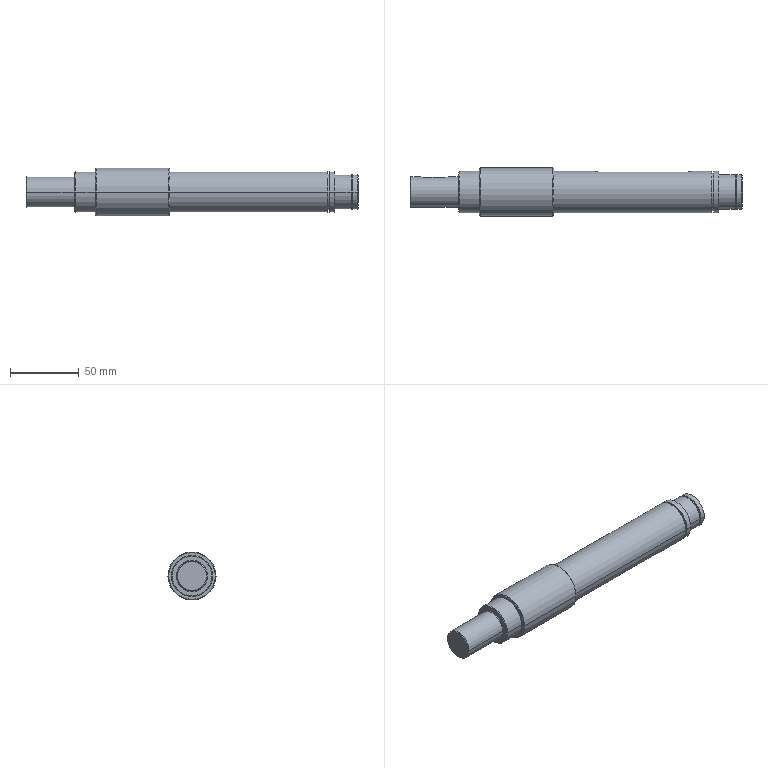Component | SolidWorks | LowerSideBeltXG-XG1-1_DrivePulleyDriveShaftXG-XG1-1 | 1 solid | 56 faces | box 241.5 x 35 x 35 mm | volume 165623 mm3 | cylinder 26 | plane 16 | cone 12 | torus 2 | commonest cylinder face diameters 30 x6 6 x5 25 x4 8 x3 22 x2 35 x2 27 x2 22.6 x2
build123d program:
from build123d import *

# Parameters (mm, degrees)
CUT_EXTRUDE2_DEPTH            = 4.5
CHAMFER1_SIZE                 = 0.5
CHAMFER3_SIZE                 = 0.5
CUT_EXTRUDE4_DEPTH            = 4
CHAMFER4_SIZE                 = 0.5
FILLET1_R                     = 0.5
CHAMFER5_SIZE                 = 0.5
CHAMFER6_SIZE                 = 0.5
SIZE_MM_DOWEL_PIN_HOLE1_D     = 6
SIZE_MM_DOWEL_PIN_HOLE1_DEPTH = 15
SIZE_MM_DOWEL_PIN_HOLE1_TIP   = 1.803


with BuildPart() as part:
    # Sketch1 → Revolve1 (revolve)
    with BuildSketch(Plane.XY, mode=Mode.PRIVATE) as revolve1_sk:
        Polygon((0, 0), (0, 12.5), (3.8, 12.5), (3.8, 11.3), (5, 11.3), (5, 12.5), (17, 12.5), (17, 15), (20.7, 15), (20.7, 13.5), (22, 13.5), (22, 15), (137, 15), (137, 17.5), (191, 17.5), (191, 15), (206, 15), (206, 11), (241.5, 11), (241.5, 0), align=None)
    revolve(revolve1_sk.sketch.rotate(Axis((-432.237, 0, 0), (1, 0, 0)), 90), axis=Axis((-432.237, 0, 0), (1, 0, 0)))

    # Sketch3 → Cut-Extrude2 (cut)
    with BuildSketch(Plane.XY.offset(15)):
        with BuildLine():
            Line((41, 4), (103, 4))
            ThreePointArc((103, 4), (107, 0), (103, -4))
            Line((103, -4), (41, -4))
            ThreePointArc((41, -4), (37, 0), (41, 4))
        make_face()
    extrude(amount=-CUT_EXTRUDE2_DEPTH, mode=Mode.SUBTRACT)

    # Chamfer1
    chamfer1_edges = [part.edges().sort_by_distance(p)[0] for p in [
        (241.5, 0, -11),
    ]]
    chamfer(chamfer1_edges, length=CHAMFER1_SIZE)

    # Chamfer3
    chamfer3_edges = [part.edges().sort_by_distance(p)[0] for p in [
        (137, 0, -17.5),
    ]]
    chamfer(chamfer3_edges, length=CHAMFER3_SIZE)

    # Sketch5 → Cut-Extrude4 (cut)
    with BuildSketch(Plane.XY.offset(11)):
        with BuildLine():
            Line((216.5, 3), (231.5, 3))
            ThreePointArc((231.5, 3), (234.5, 0), (231.5, -3))
            Line((231.5, -3), (216.5, -3))
            ThreePointArc((216.5, -3), (213.5, 0), (216.5, 3))
        make_face()
    extrude(amount=-CUT_EXTRUDE4_DEPTH, mode=Mode.SUBTRACT)

    # Chamfer4
    chamfer4_edges = [part.edges().sort_by_distance(p)[0] for p in [
        (0, 0, -12.5),
    ]]
    chamfer(chamfer4_edges, length=CHAMFER4_SIZE)

    # Fillet1
    fillet1_edges = [part.edges().sort_by_distance(p)[0] for p in [
        (206, 0, -11),
    ]]
    fillet(fillet1_edges, radius=FILLET1_R)

    # Chamfer5
    chamfer5_edges = [part.edges().sort_by_distance(p)[0] for p in [
        (191, 0, -17.5),
    ]]
    chamfer(chamfer5_edges, length=CHAMFER5_SIZE)

    # Chamfer6
    chamfer6_edges = [part.edges().sort_by_distance(p)[0] for p in [
        (206, 0, -15),
    ]]
    chamfer(chamfer6_edges, length=CHAMFER6_SIZE)

    # Size mm Dowel Pin Hole1
    with Locations(Plane.ZY):
        with Locations((0, 0)):
            Hole(SIZE_MM_DOWEL_PIN_HOLE1_D / 2, depth=SIZE_MM_DOWEL_PIN_HOLE1_DEPTH)
            with Locations((0, 0, -(SIZE_MM_DOWEL_PIN_HOLE1_DEPTH + SIZE_MM_DOWEL_PIN_HOLE1_TIP / 2))):  # 118° drill point
                Cone(0, SIZE_MM_DOWEL_PIN_HOLE1_D / 2, SIZE_MM_DOWEL_PIN_HOLE1_TIP, mode=Mode.SUBTRACT)


solid = part.part

# Placed as in the assembly
solid = solid.moved(Location((-179.22, 625, 114), (-90, 0, 180)))